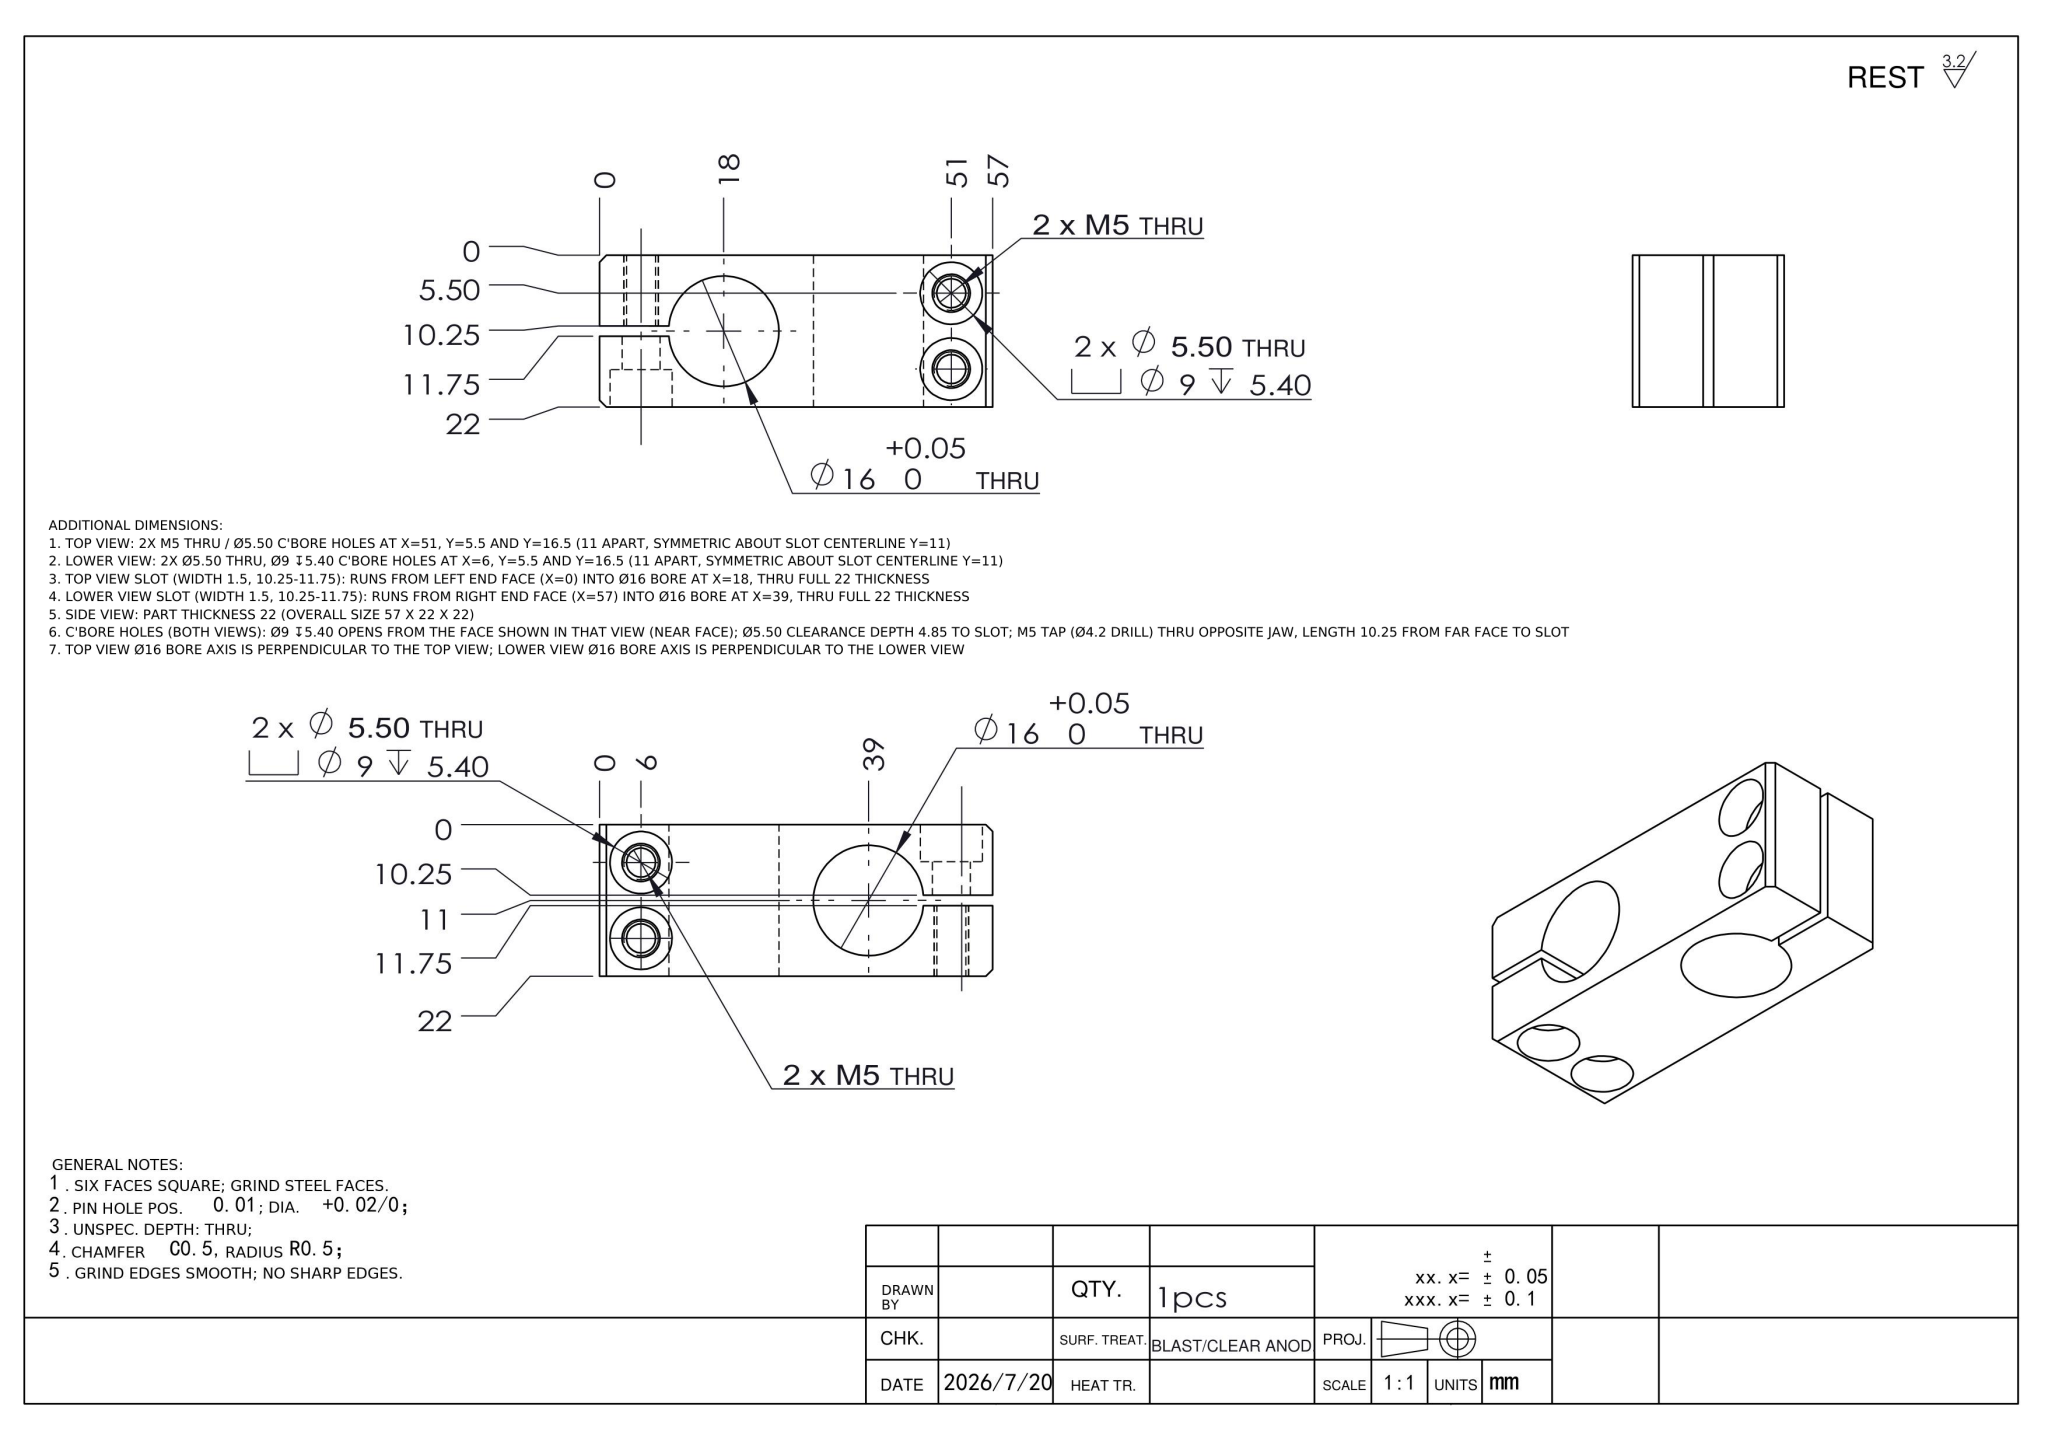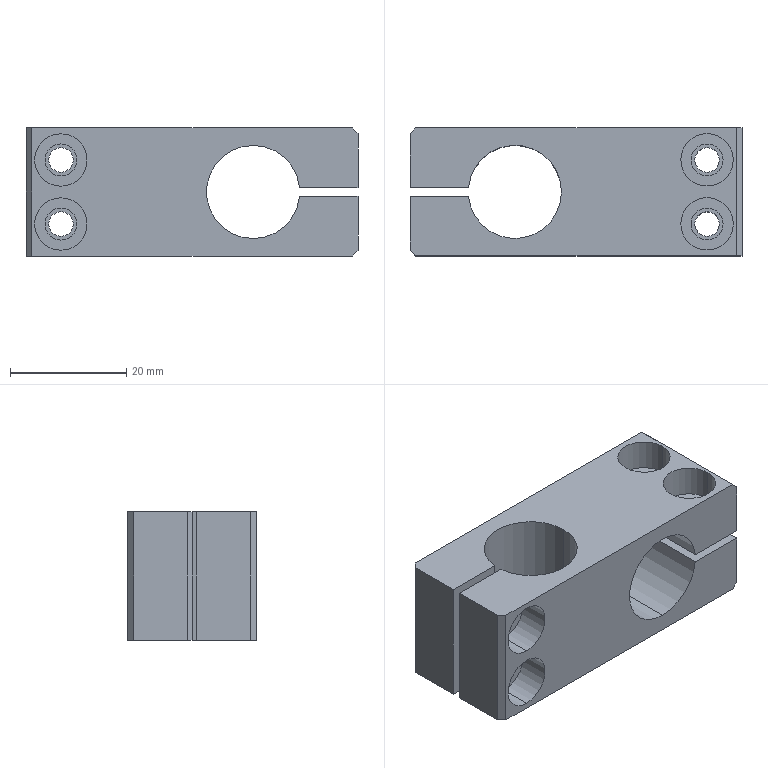Part | NX | mm | 1 solid | 49 faces | box 57 x 22 x 22 mm | volume 15633 mm3 | cylinder 29 | plane 20 | commonest cylinder face diameters 4.2 x8 9 x8 5.5 x8 16 x5